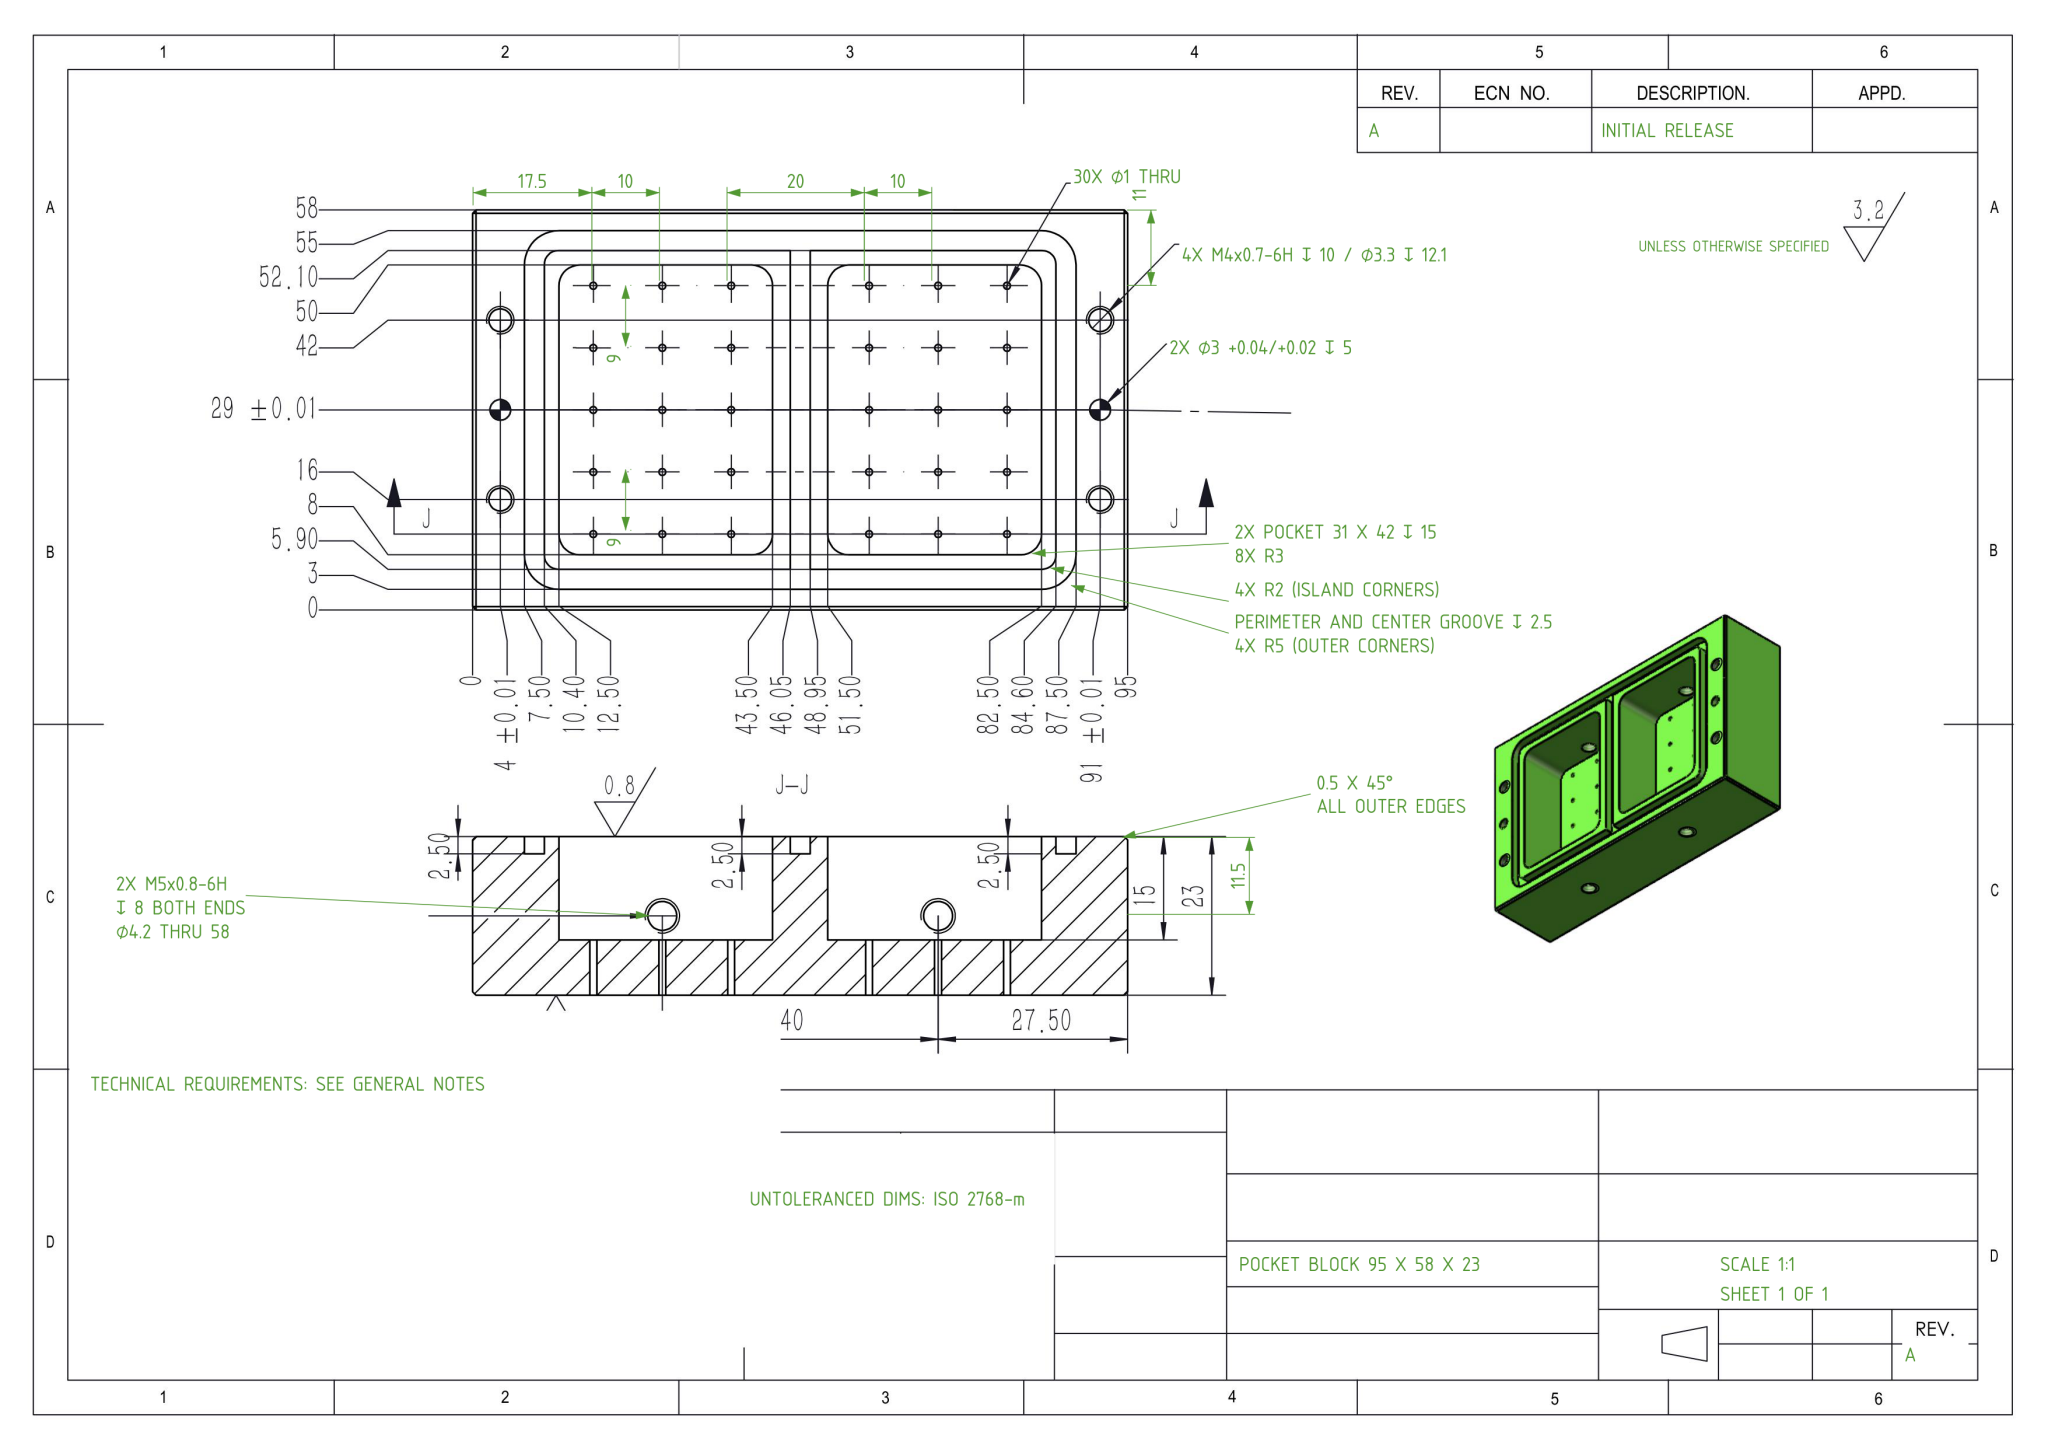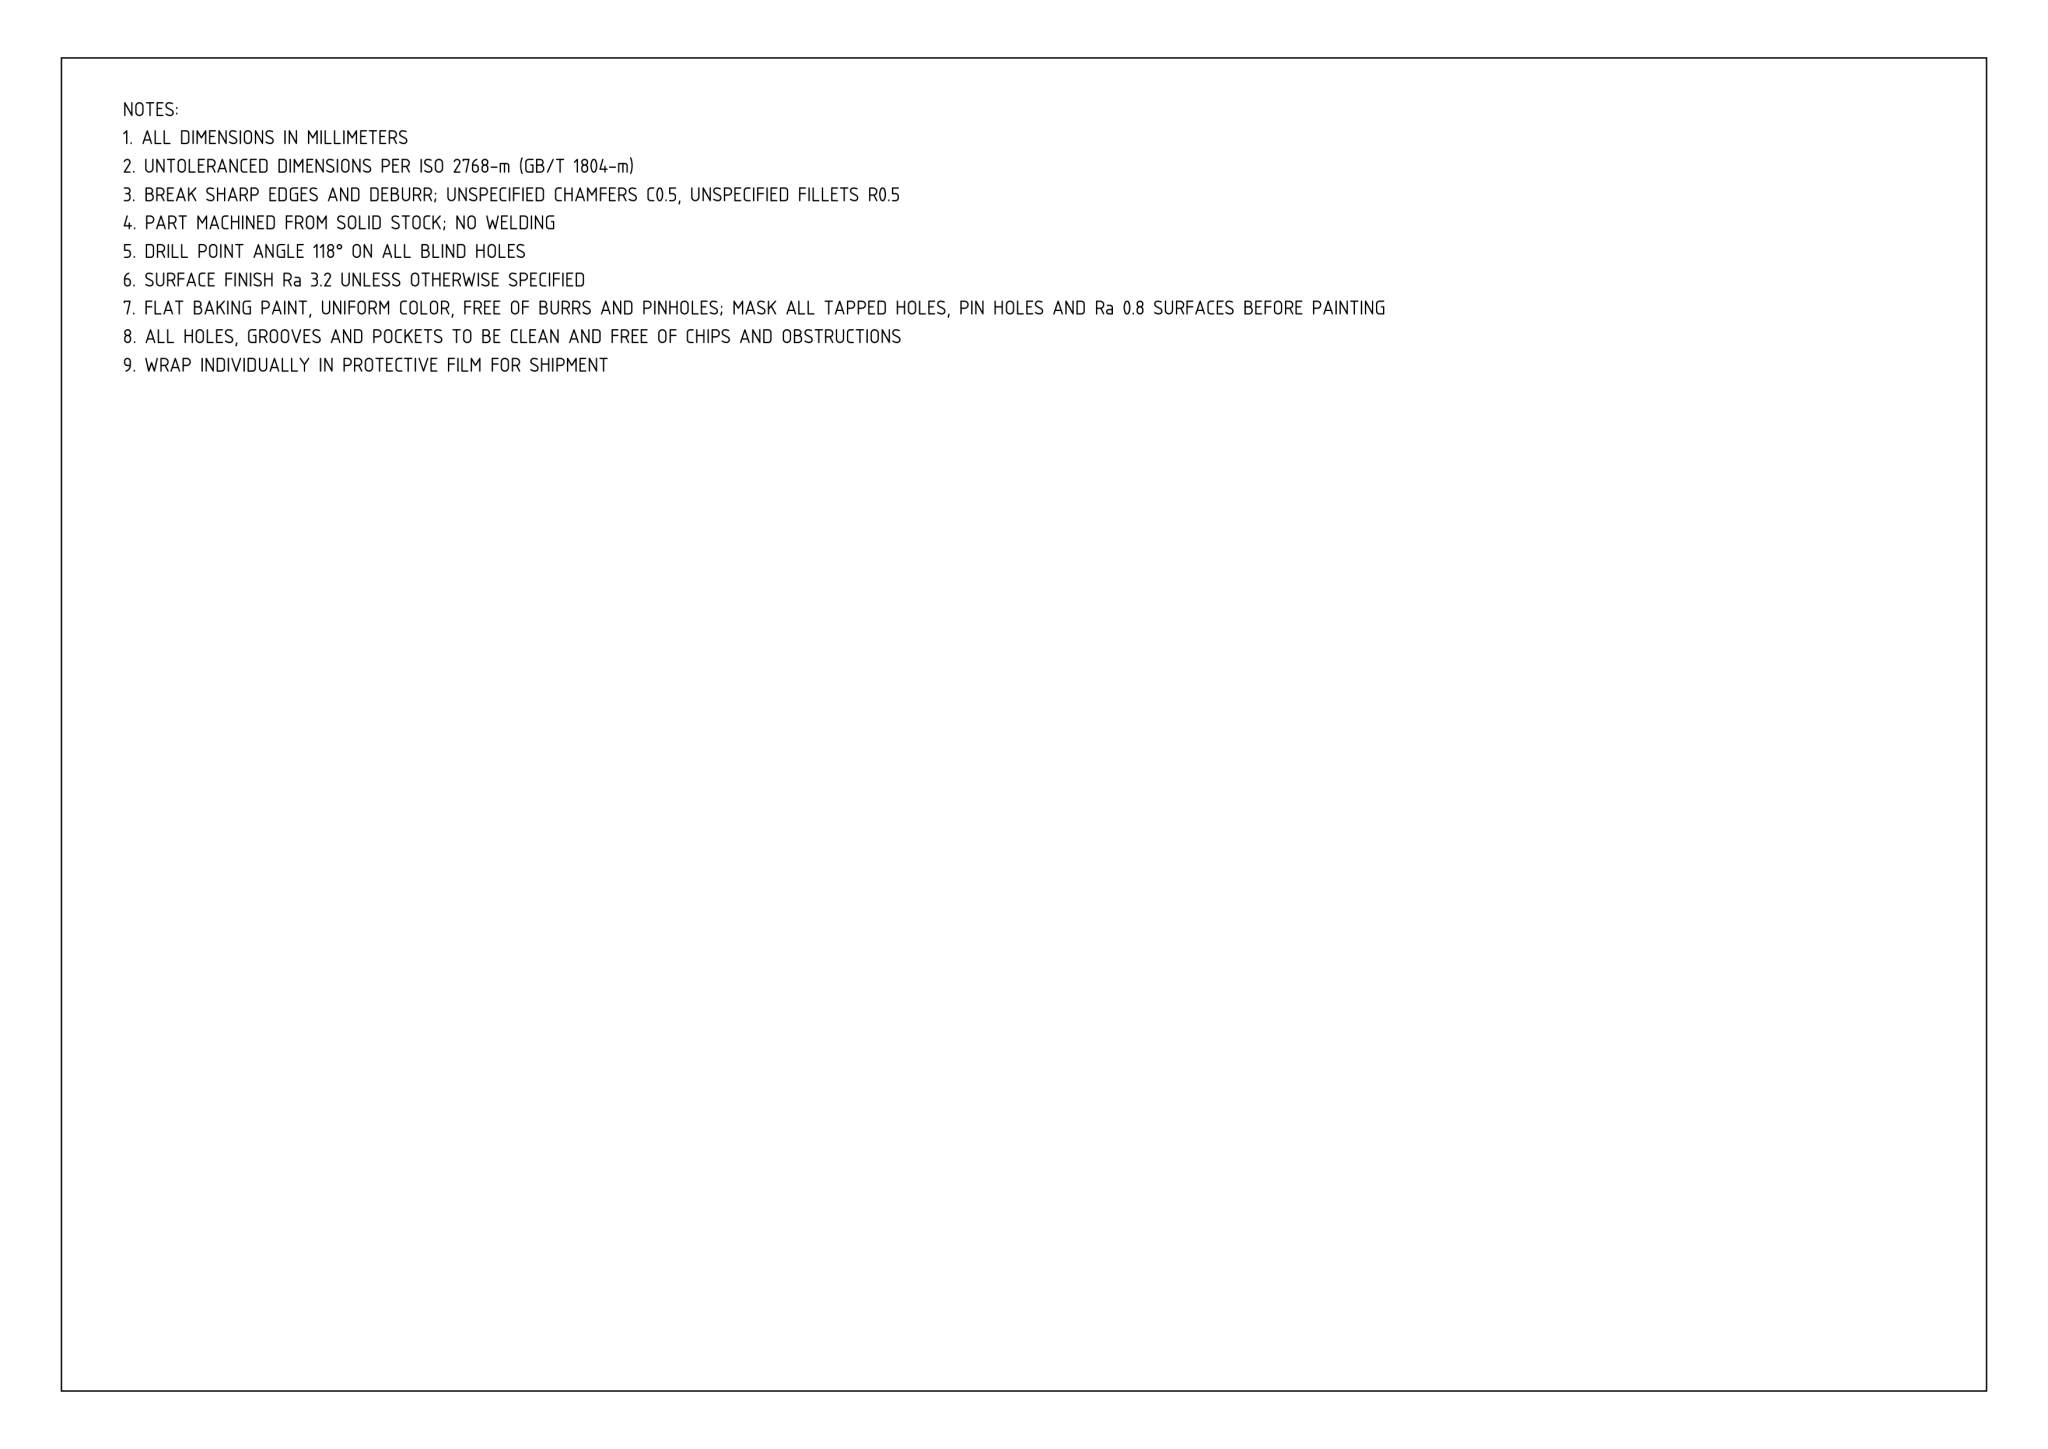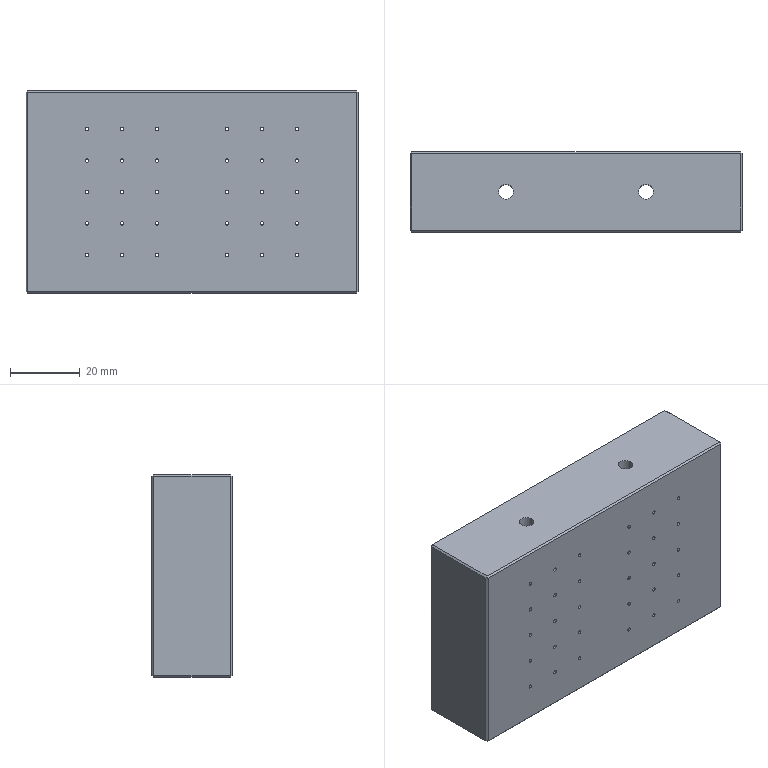Part | NX | mm | 1 solid | 159 faces | box 95 x 23 x 58 mm | volume 84563 mm3 | cylinder 96 | plane 51 | cone 12 | commonest cylinder face diameters 1 x60 3.3 x8 4.2 x8 6 x8 3 x4 10 x4 4 x4